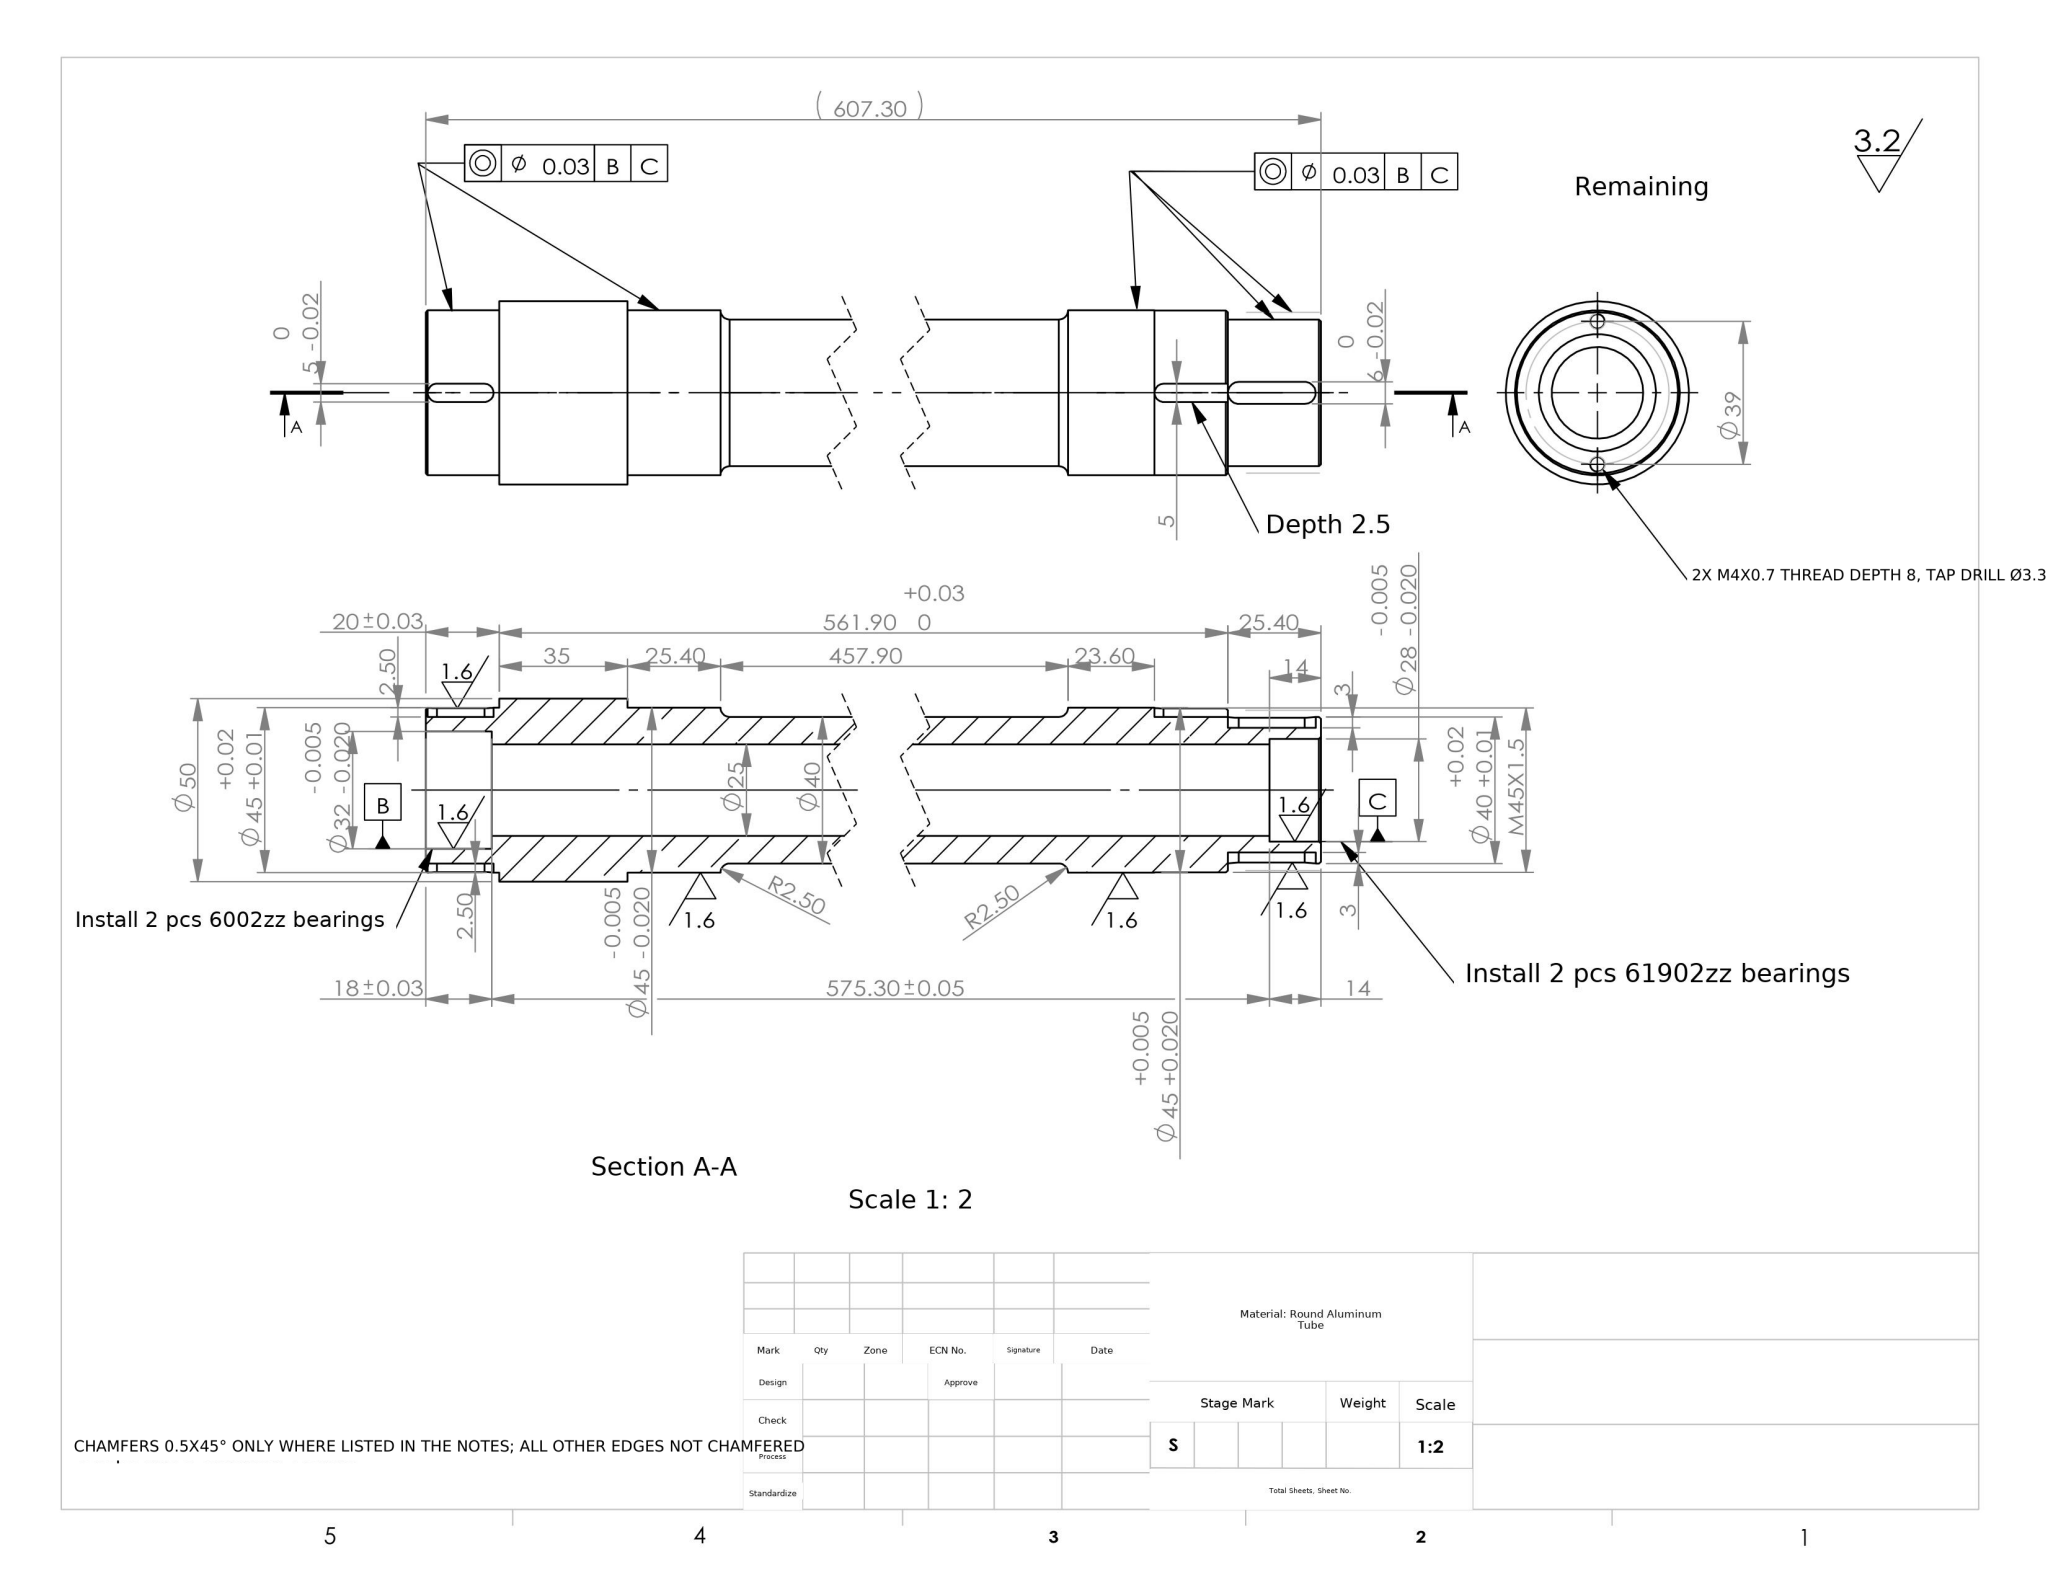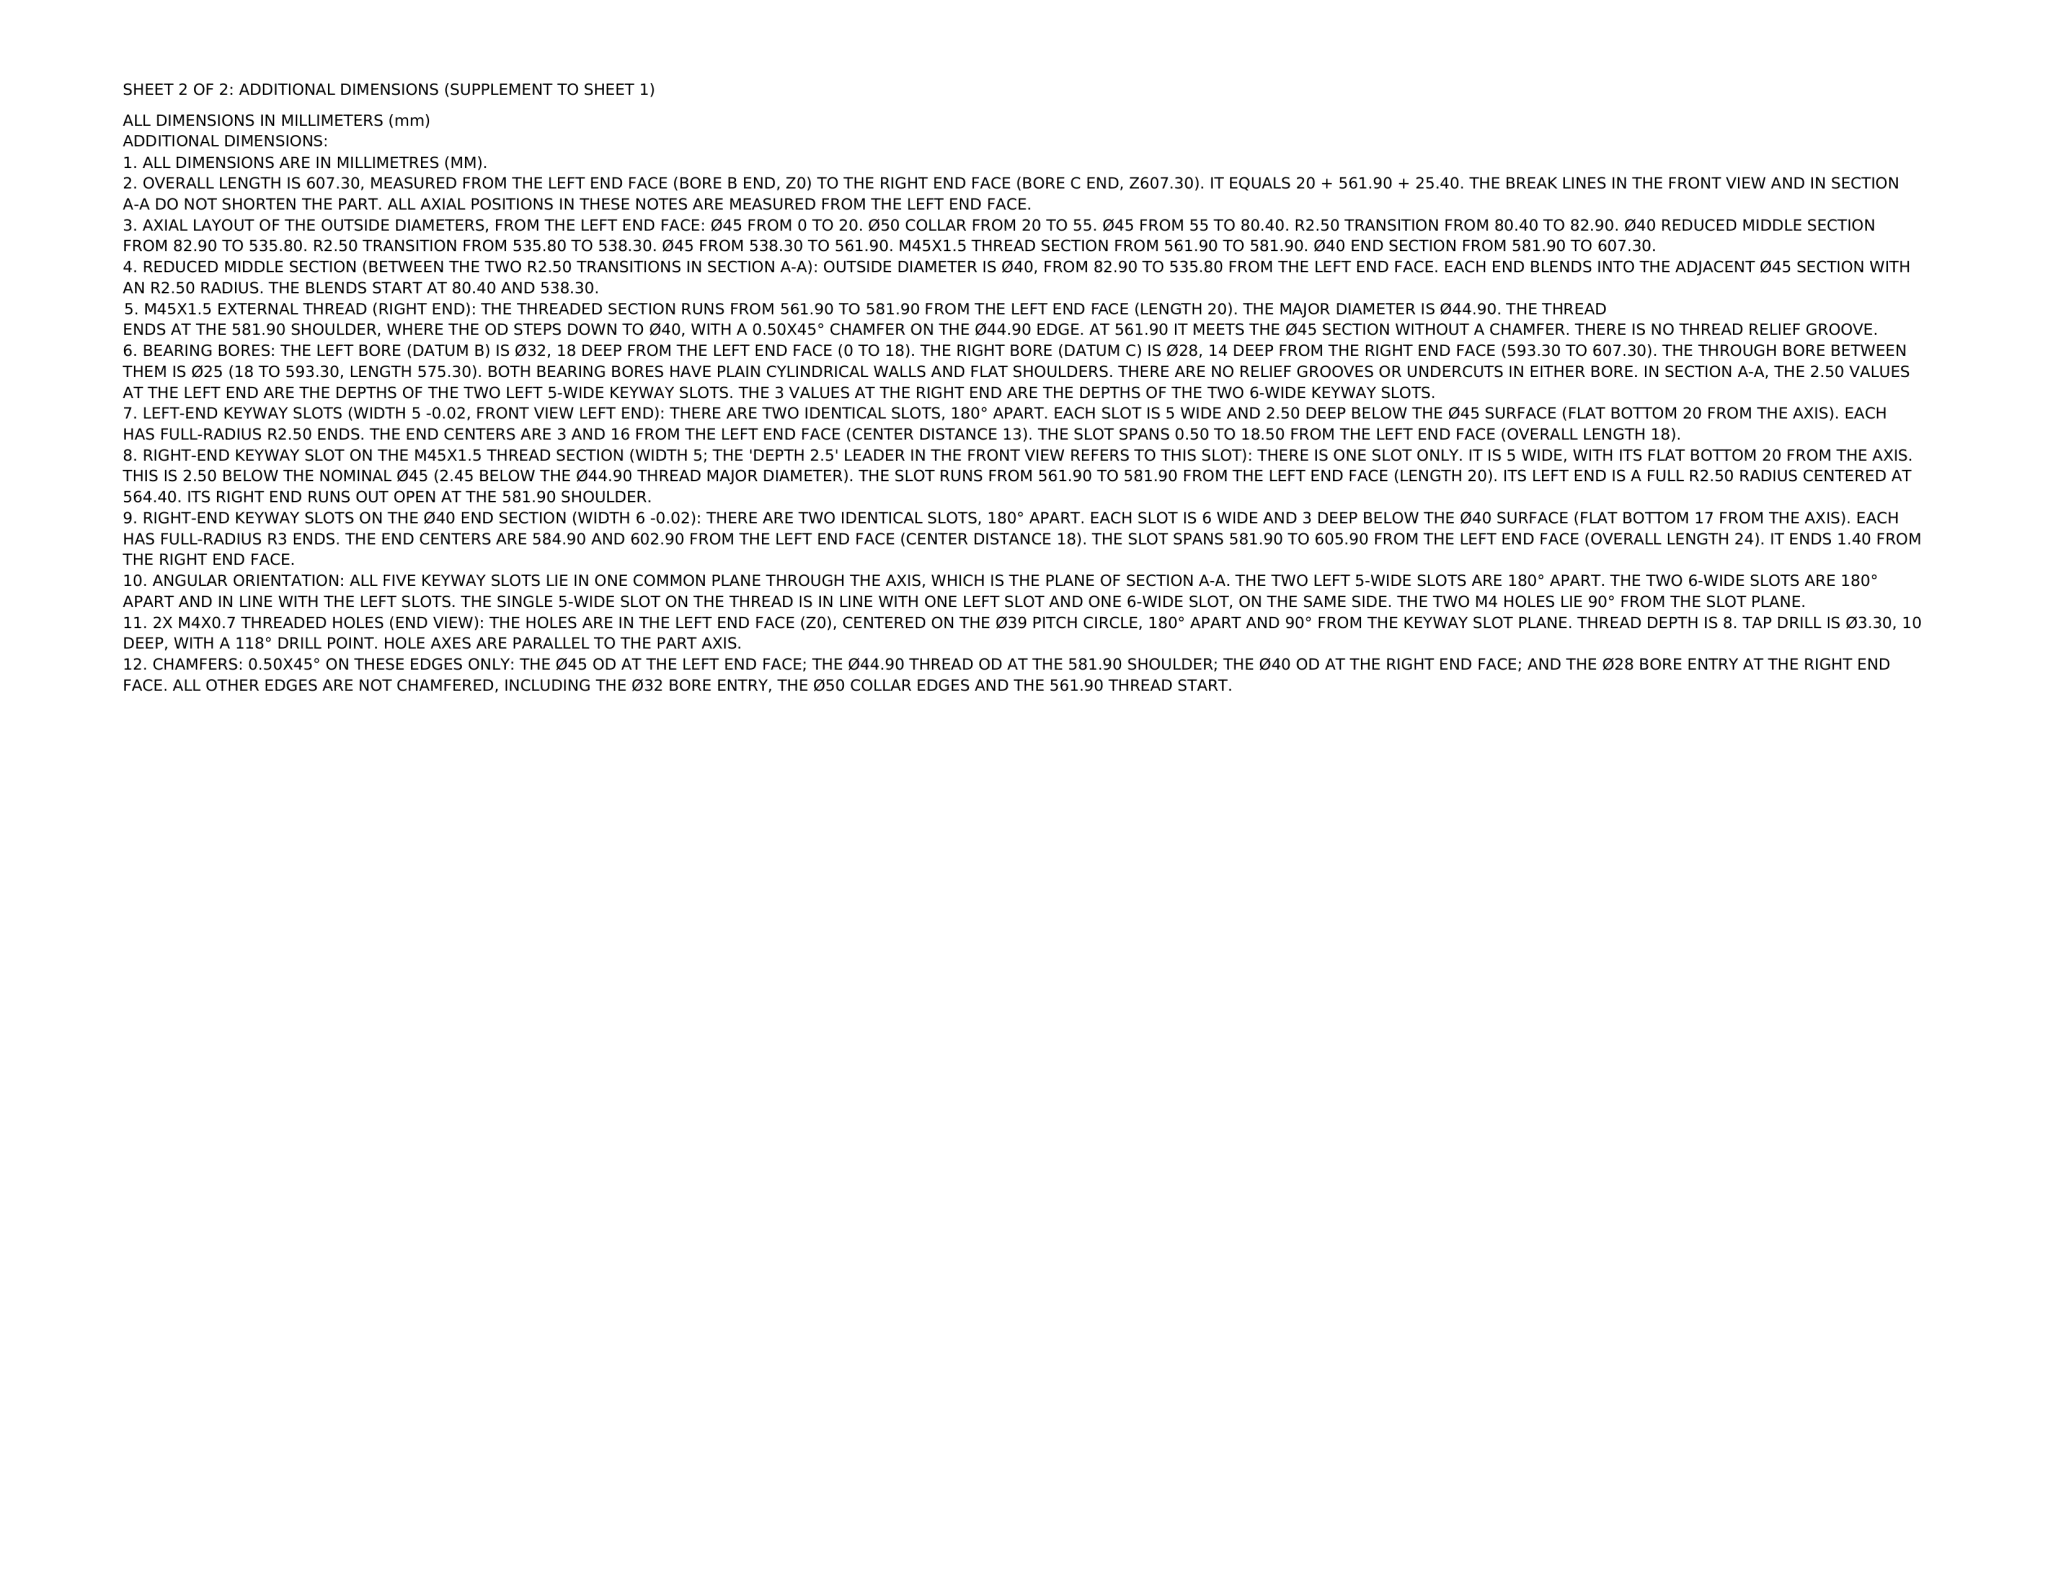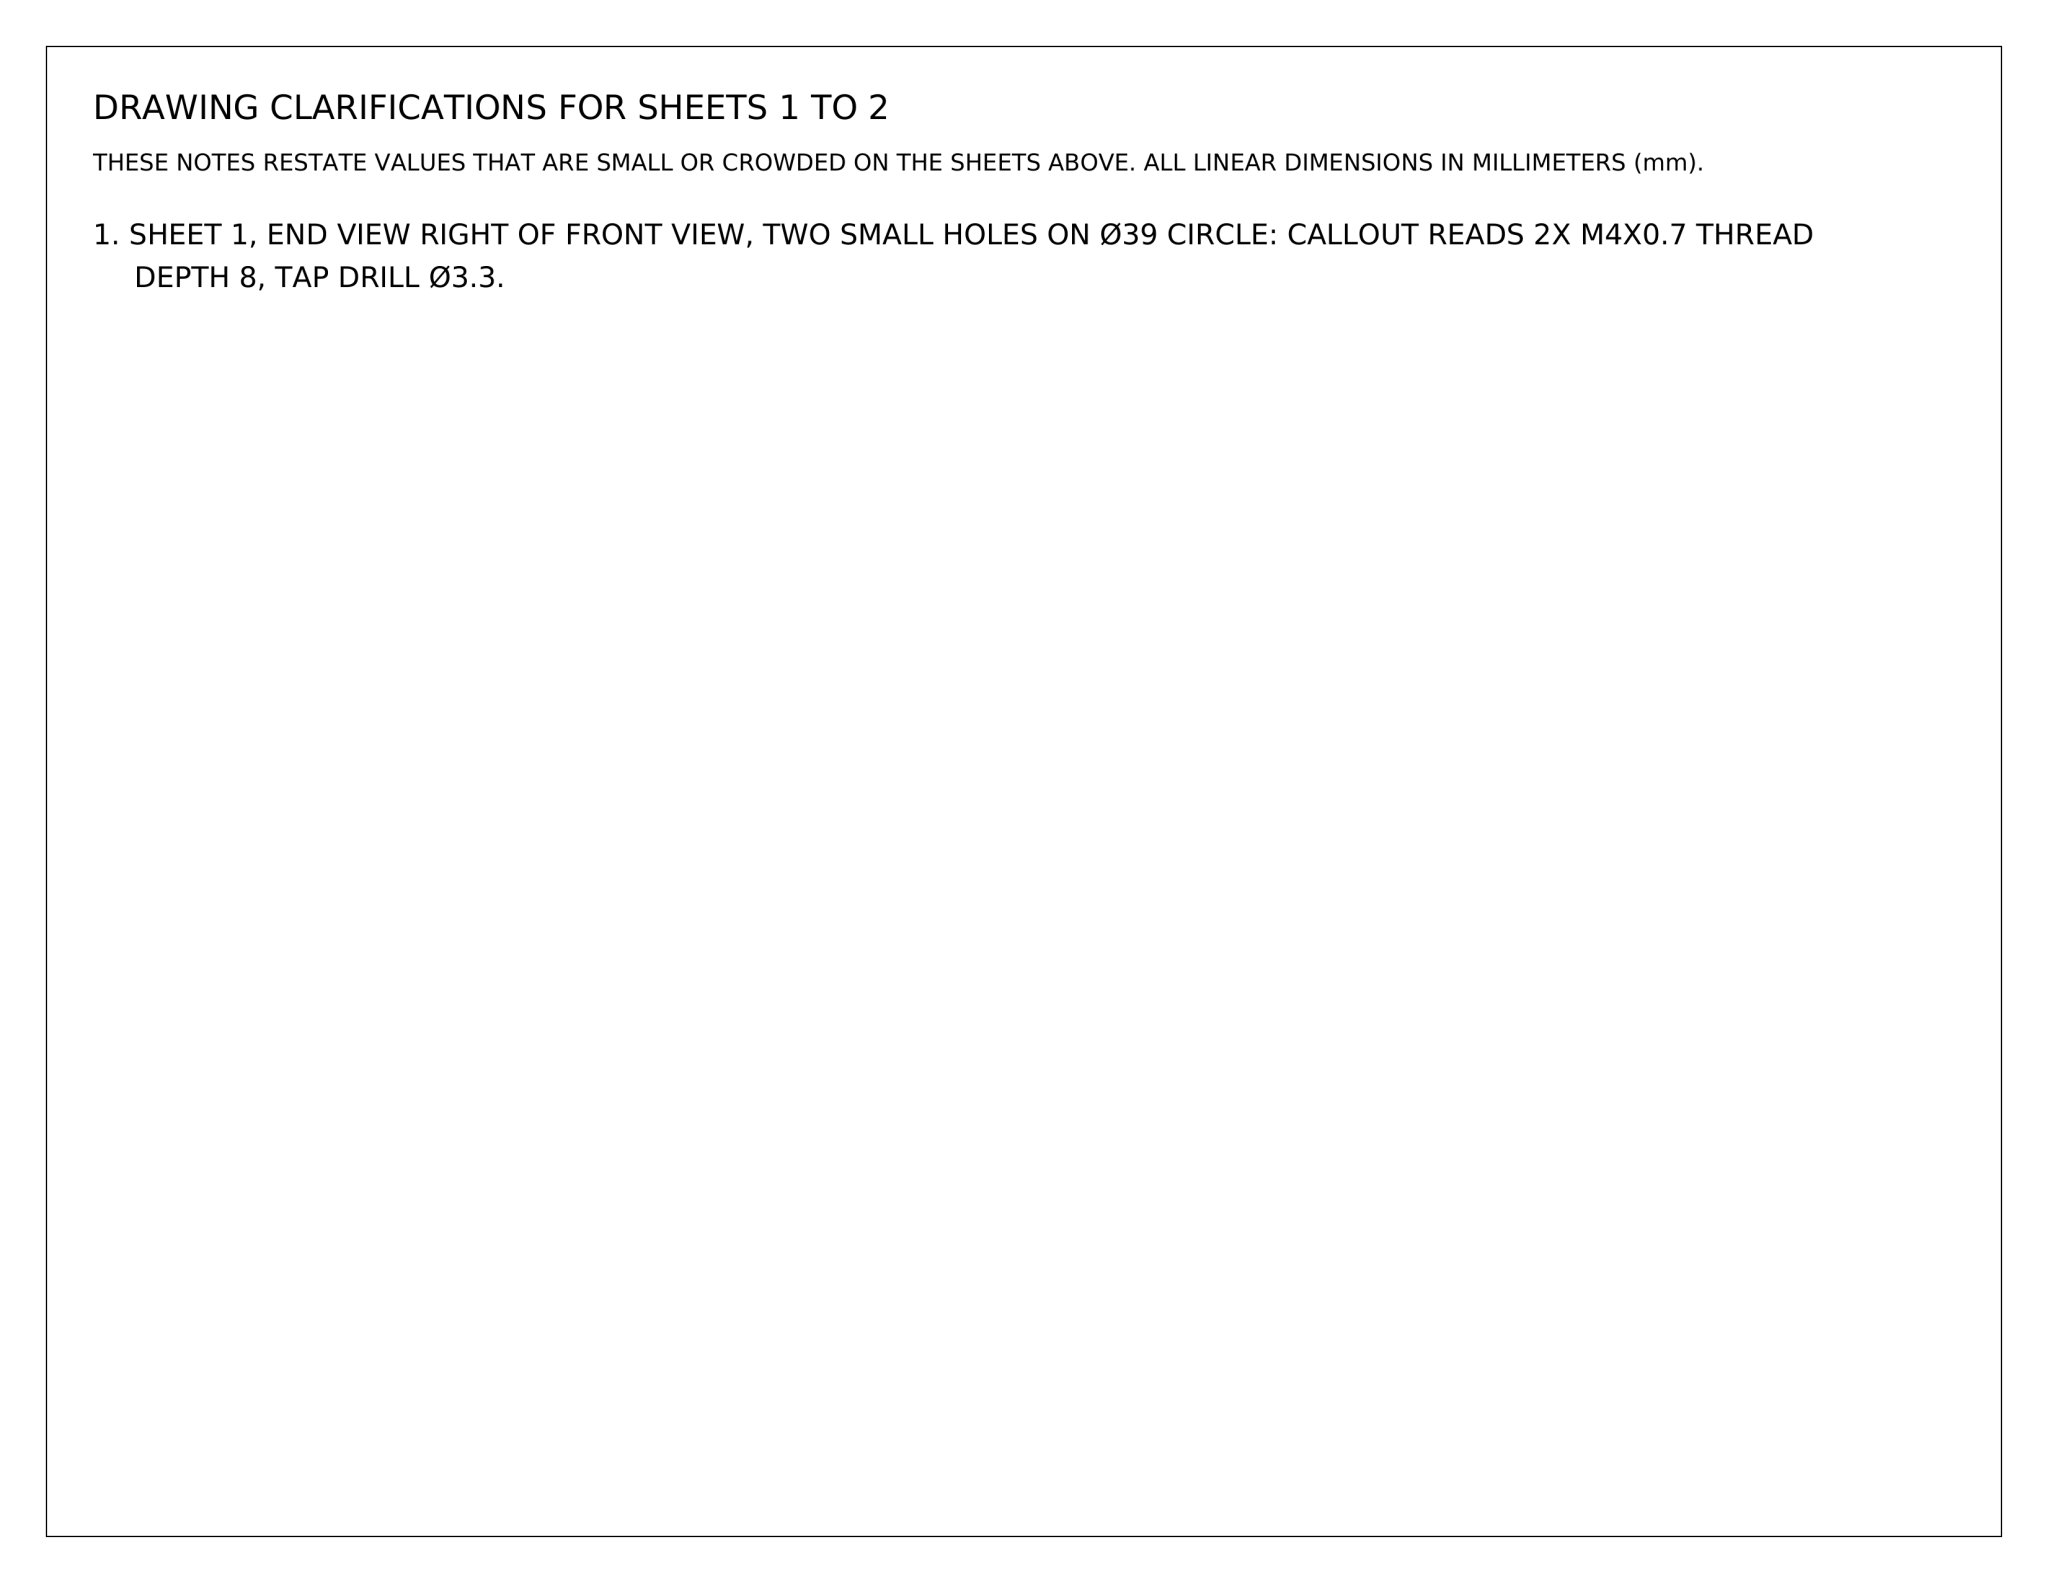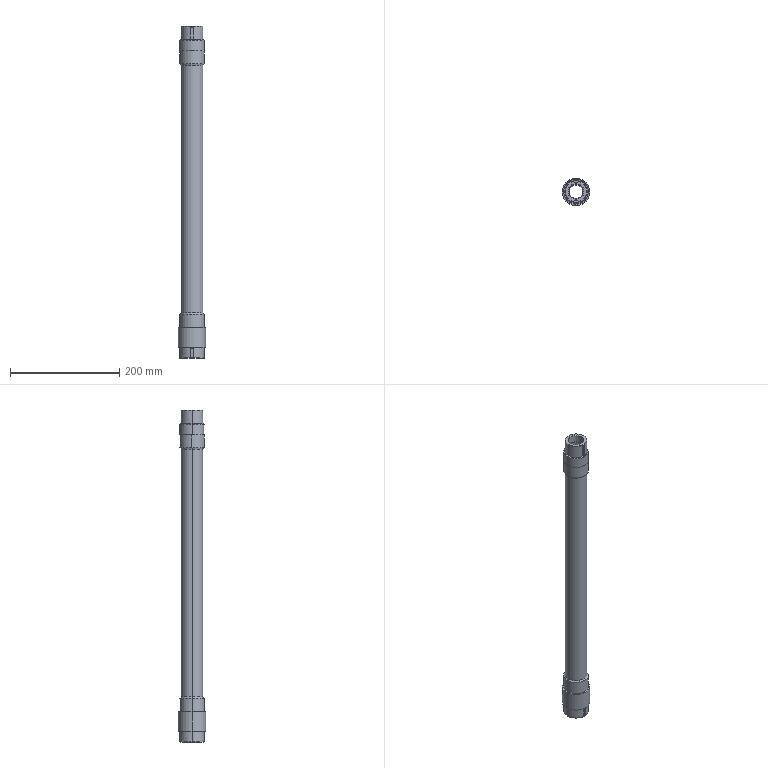Part | NX | mm | 1 solid | 74 faces | box 50 x 50 x 607.3 mm | volume 510552 mm3 | cylinder 36 | plane 25 | cone 9 | torus 4 | commonest cylinder face diameters 45 x6 5 x6 6 x5 40 x4 4 x4 44.9 x3 28 x2 50 x2